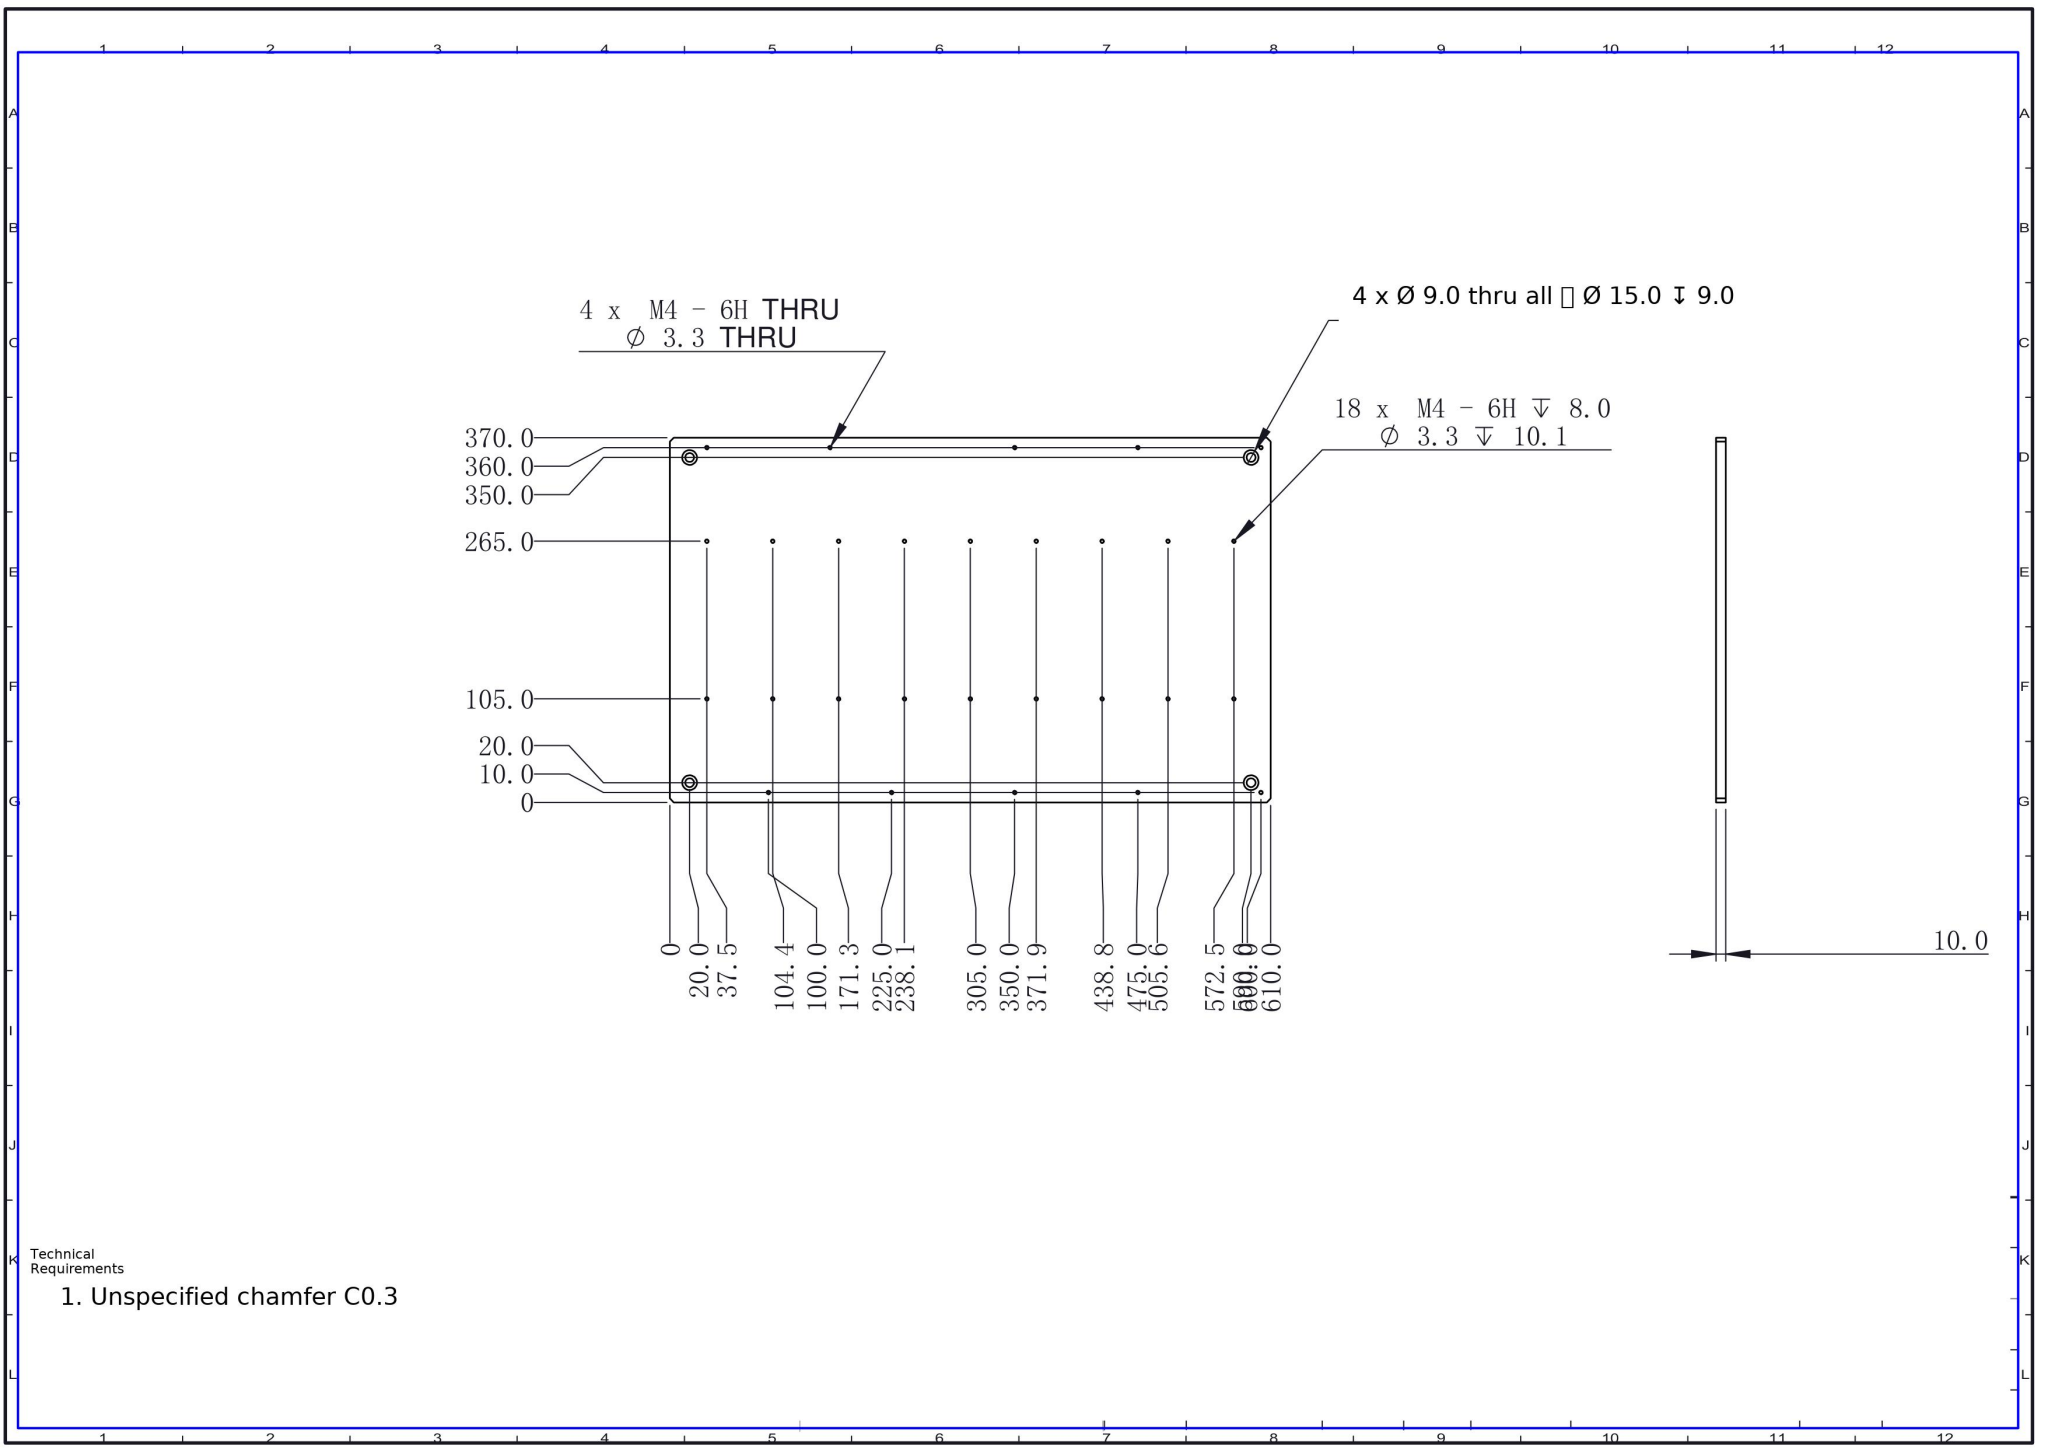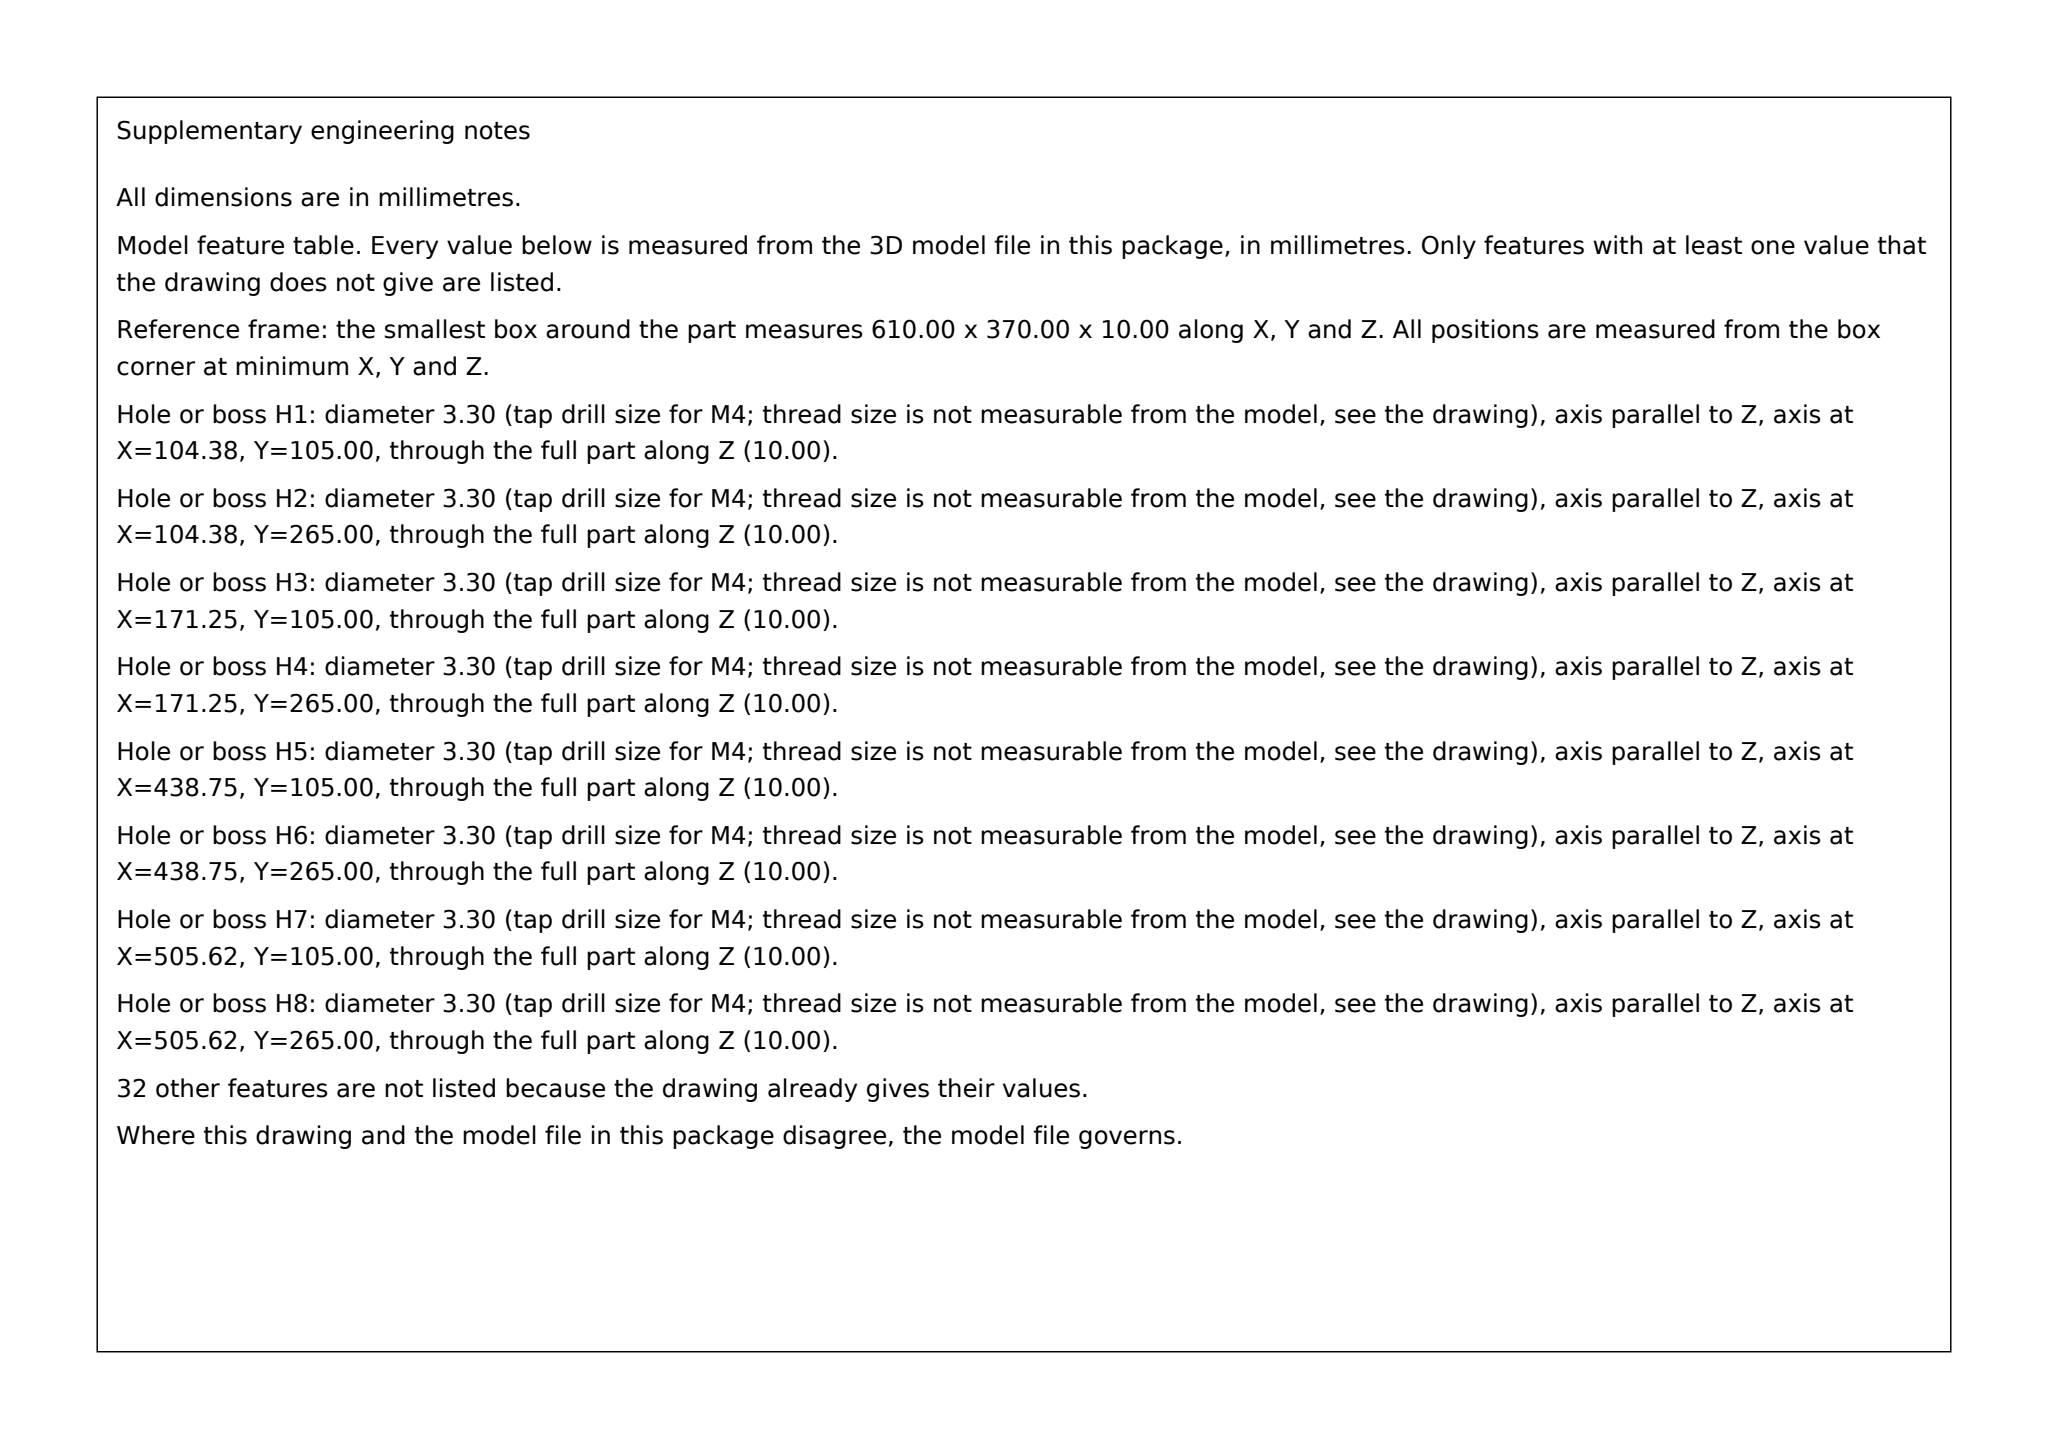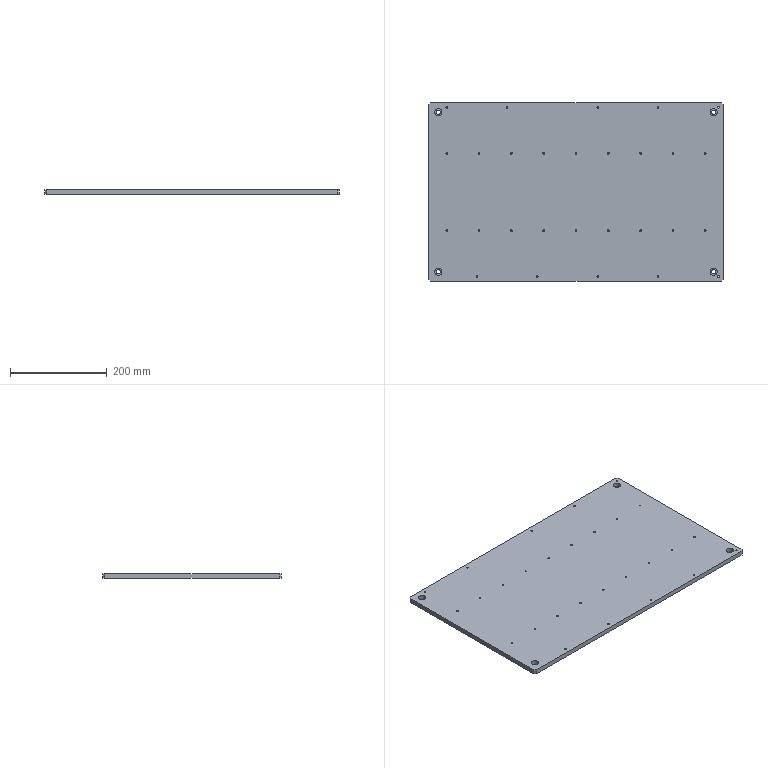Part | SolidWorks | mm | 1 solid | 86 faces | box 610 x 370 x 10 mm | volume 2247669 mm3 | cylinder 72 | plane 14 | commonest cylinder face diameters 3.3 x56 15 x8 9 x8
build123d program:
from build123d import *

# Parameters (mm, degrees)
SKETCH1_W                                         = 610
SKETCH1_H                                         = 370
BOSS_EXTRUDE1_DEPTH                               = 5
HOLE_SIZE_ACCORDING_TO_HEXAGON_SOCKET_D           = 9
HOLE_SIZE_ACCORDING_TO_HEXAGON_SOCKET_CBORE_D     = 15
HOLE_SIZE_ACCORDING_TO_HEXAGON_SOCKET_CBORE_DEPTH = 9
M4_TAPPED_HOLE1_D                                 = 3.3
CHAMFER1_SIZE                                     = 4
M4_TAPPED_HOLE2_D                                 = 3.3
M4_TAPPED_HOLE3_D                                 = 3.3
M4_TAPPED_HOLE3_DEPTH                             = 10.1
M4_TAPPED_HOLE3_TIP                               = 0.9914


with BuildPart() as part:
    # Sketch1 → Boss-Extrude1 (new, symmetric)
    with BuildSketch(Plane.XY):
        Rectangle(SKETCH1_W, SKETCH1_H)
    extrude(amount=BOSS_EXTRUDE1_DEPTH, both=True)

    # Hole Size _ according to_ Hexagon Socket (through all)
    with Locations(Plane.XY.offset(5)):
        with Locations((-285, 165), (-285, -165), (285, -165), (285, 165)):
            CounterBoreHole(HOLE_SIZE_ACCORDING_TO_HEXAGON_SOCKET_D / 2, HOLE_SIZE_ACCORDING_TO_HEXAGON_SOCKET_CBORE_D / 2, HOLE_SIZE_ACCORDING_TO_HEXAGON_SOCKET_CBORE_DEPTH)

    # M4 Tapped Hole1 (through all)
    with Locations(Plane.XY.offset(5)):
        with Locations((-142.5, 175), (-267.5, 175), (-205, -175), (-80, -175)):
            Hole(M4_TAPPED_HOLE1_D / 2)

    # Chamfer1
    chamfer1_edges = [part.edges().sort_by_distance(p)[0] for p in [
        (-305, 185, 0),
        (305, 185, 0),
        (305, -185, 0),
        (-305, -185, 0),
    ]]
    chamfer(chamfer1_edges, length=CHAMFER1_SIZE)

    # M4 Tapped Hole2 (through all)
    with Locations(Plane.XY.offset(5)):
        with Locations((45, -175), (170, -175), (295, -175), (295, 175), (170, 175), (45, 175)):
            Hole(M4_TAPPED_HOLE2_D / 2)

    # M4 Tapped Hole3
    with Locations(Plane.XY.offset(5)):
        with Locations((-267.5, 80), (-200.625, 80), (-133.75, 80), (-66.875, 80), (0, 80), (66.875, 80), (133.75, 80), (200.625, 80), (267.5, 80), (-200.625, -80), (-133.75, -80), (-66.875, -80), (0, -80), (66.875, -80), (133.75, -80), (200.625, -80), (267.5, -80), (-267.5, -80)):
            Hole(M4_TAPPED_HOLE3_D / 2, depth=M4_TAPPED_HOLE3_DEPTH)
            with Locations((0, 0, -(M4_TAPPED_HOLE3_DEPTH + M4_TAPPED_HOLE3_TIP / 2))):  # 118° drill point
                Cone(0, M4_TAPPED_HOLE3_D / 2, M4_TAPPED_HOLE3_TIP, mode=Mode.SUBTRACT)


solid = part.part